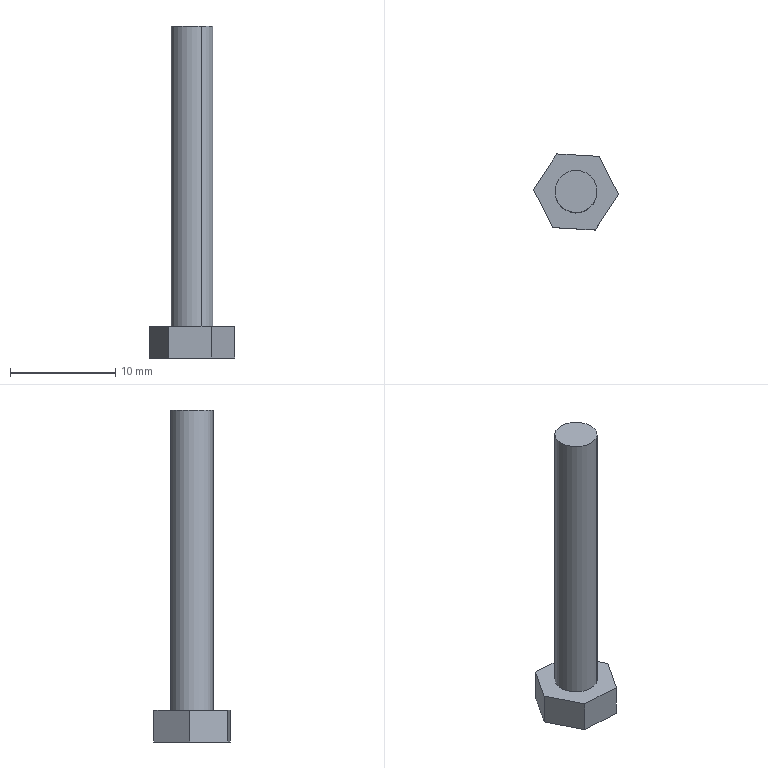Component | SolidWorks | 4Bolt-3 | 1 solid | 11 faces | box 8.07 x 7.22 x 31.5 mm | volume 485 mm3 | plane 9 | cylinder 2 | commonest cylinder face diameters 4 x2
STEP:
#1=COLOUR_RGB('',0.7922,0.8196,0.9333);
#2=FILL_AREA_STYLE_COLOUR('',#1);
#3=FILL_AREA_STYLE('',(#2));
#4=SURFACE_STYLE_FILL_AREA(#3);
#5=SURFACE_SIDE_STYLE('',(#4));
#6=SURFACE_STYLE_USAGE(.BOTH.,#5);
#7=PRESENTATION_STYLE_ASSIGNMENT((#6));
#8=CARTESIAN_POINT('',(4.312,4.161,2.255));
#9=VERTEX_POINT('',#8);
#10=CARTESIAN_POINT('',(4.241,4.302,2.255));
#11=VERTEX_POINT('',#10);
#12=CARTESIAN_POINT('',(4.277,4.231,2.255));
#13=DIRECTION('',(0.,0.,1.));
#14=DIRECTION('',(0.4489,-0.8936,0.));
#15=AXIS2_PLACEMENT_3D('',#12,#13,#14);
#16=CIRCLE('',#15,0.07874);
#17=EDGE_CURVE('',#9,#11,#16,.T.);
#18=ORIENTED_EDGE('',*,*,#17,.F.);
#19=CARTESIAN_POINT('',(4.312,4.161,1.133));
#20=VERTEX_POINT('',#19);
#21=CARTESIAN_POINT('',(4.312,4.161,2.255));
#22=DIRECTION('',(0.,0.,-1.));
#23=VECTOR('',#22,39.37);
#24=LINE('',#21,#23);
#25=EDGE_CURVE('',#9,#20,#24,.T.);
#26=ORIENTED_EDGE('',*,*,#25,.T.);
#27=CARTESIAN_POINT('',(4.241,4.302,1.133));
#28=VERTEX_POINT('',#27);
#29=CARTESIAN_POINT('',(4.277,4.231,1.133));
#30=DIRECTION('',(0.,0.,1.));
#31=DIRECTION('',(0.4489,-0.8936,0.));
#32=AXIS2_PLACEMENT_3D('',#29,#30,#31);
#33=CIRCLE('',#32,0.07874);
#34=EDGE_CURVE('',#20,#28,#33,.T.);
#35=ORIENTED_EDGE('',*,*,#34,.T.);
#36=CARTESIAN_POINT('',(4.241,4.302,2.255));
#37=DIRECTION('',(0.,0.,-1.));
#38=VECTOR('',#37,39.37);
#39=LINE('',#36,#38);
#40=EDGE_CURVE('',#11,#28,#39,.T.);
#41=ORIENTED_EDGE('',*,*,#40,.F.);
#42=EDGE_LOOP('',(#18,#26,#35,#41));
#43=FACE_OUTER_BOUND('',#42,.T.);
#44=CARTESIAN_POINT('',(4.277,4.231,2.255));
#45=DIRECTION('',(0.,0.,-1.));
#46=DIRECTION('',(-0.4489,0.8936,0.));
#47=AXIS2_PLACEMENT_3D('',#44,#45,#46);
#48=CYLINDRICAL_SURFACE('',#47,0.07874);
#49=ADVANCED_FACE('',(#43),#48,.T.);
#50=CARTESIAN_POINT('',(4.189,4.098,1.015));
#51=VERTEX_POINT('',#50);
#52=CARTESIAN_POINT('',(4.348,4.089,1.015));
#53=VERTEX_POINT('',#52);
#54=CARTESIAN_POINT('',(4.189,4.098,1.015));
#55=DIRECTION('',(0.9983,-0.05809,0.));
#56=VECTOR('',#55,39.37);
#57=LINE('',#54,#56);
#58=EDGE_CURVE('',#51,#53,#57,.T.);
#59=ORIENTED_EDGE('',*,*,#58,.T.);
#60=CARTESIAN_POINT('',(4.348,4.089,1.133));
#61=VERTEX_POINT('',#60);
#62=CARTESIAN_POINT('',(4.348,4.089,1.133));
#63=DIRECTION('',(0.,0.,-1.));
#64=VECTOR('',#63,39.37);
#65=LINE('',#62,#64);
#66=EDGE_CURVE('',#61,#53,#65,.T.);
#67=ORIENTED_EDGE('',*,*,#66,.F.);
#68=CARTESIAN_POINT('',(4.189,4.098,1.133));
#69=VERTEX_POINT('',#68);
#70=CARTESIAN_POINT('',(4.189,4.098,1.133));
#71=DIRECTION('',(0.9983,-0.05809,0.));
#72=VECTOR('',#71,39.37);
#73=LINE('',#70,#72);
#74=EDGE_CURVE('',#69,#61,#73,.T.);
#75=ORIENTED_EDGE('',*,*,#74,.F.);
#76=CARTESIAN_POINT('',(4.189,4.098,1.133));
#77=DIRECTION('',(0.,0.,-1.));
#78=VECTOR('',#77,39.37);
#79=LINE('',#76,#78);
#80=EDGE_CURVE('',#69,#51,#79,.T.);
#81=ORIENTED_EDGE('',*,*,#80,.T.);
#82=EDGE_LOOP('',(#59,#67,#75,#81));
#83=FACE_OUTER_BOUND('',#82,.T.);
#84=CARTESIAN_POINT('',(4.189,4.098,1.133));
#85=DIRECTION('',(0.05809,0.9983,0.));
#86=DIRECTION('',(-0.9983,0.05809,0.));
#87=AXIS2_PLACEMENT_3D('',#84,#85,#86);
#88=PLANE('',#87);
#89=ADVANCED_FACE('',(#83),#88,.F.);
#90=CARTESIAN_POINT('',(4.435,4.222,1.015));
#91=VERTEX_POINT('',#90);
#92=CARTESIAN_POINT('',(4.348,4.089,1.015));
#93=DIRECTION('',(0.5495,0.8355,0.));
#94=VECTOR('',#93,39.37);
#95=LINE('',#92,#94);
#96=EDGE_CURVE('',#53,#91,#95,.T.);
#97=ORIENTED_EDGE('',*,*,#96,.T.);
#98=CARTESIAN_POINT('',(4.435,4.222,1.133));
#99=VERTEX_POINT('',#98);
#100=CARTESIAN_POINT('',(4.435,4.222,1.133));
#101=DIRECTION('',(0.,0.,-1.));
#102=VECTOR('',#101,39.37);
#103=LINE('',#100,#102);
#104=EDGE_CURVE('',#99,#91,#103,.T.);
#105=ORIENTED_EDGE('',*,*,#104,.F.);
#106=CARTESIAN_POINT('',(4.348,4.089,1.133));
#107=DIRECTION('',(0.5495,0.8355,0.));
#108=VECTOR('',#107,39.37);
#109=LINE('',#106,#108);
#110=EDGE_CURVE('',#61,#99,#109,.T.);
#111=ORIENTED_EDGE('',*,*,#110,.F.);
#112=ORIENTED_EDGE('',*,*,#66,.T.);
#113=EDGE_LOOP('',(#97,#105,#111,#112));
#114=FACE_OUTER_BOUND('',#113,.T.);
#115=CARTESIAN_POINT('',(4.348,4.089,1.133));
#116=DIRECTION('',(-0.8355,0.5495,0.));
#117=DIRECTION('',(-0.5495,-0.8355,0.));
#118=AXIS2_PLACEMENT_3D('',#115,#116,#117);
#119=PLANE('',#118);
#120=ADVANCED_FACE('',(#114),#119,.F.);
#121=CARTESIAN_POINT('',(4.364,4.364,1.015));
#122=VERTEX_POINT('',#121);
#123=CARTESIAN_POINT('',(4.435,4.222,1.015));
#124=DIRECTION('',(-0.4489,0.8936,0.));
#125=VECTOR('',#124,39.37);
#126=LINE('',#123,#125);
#127=EDGE_CURVE('',#91,#122,#126,.T.);
#128=ORIENTED_EDGE('',*,*,#127,.T.);
#129=CARTESIAN_POINT('',(4.364,4.364,1.133));
#130=VERTEX_POINT('',#129);
#131=CARTESIAN_POINT('',(4.364,4.364,1.133));
#132=DIRECTION('',(0.,0.,-1.));
#133=VECTOR('',#132,39.37);
#134=LINE('',#131,#133);
#135=EDGE_CURVE('',#130,#122,#134,.T.);
#136=ORIENTED_EDGE('',*,*,#135,.F.);
#137=CARTESIAN_POINT('',(4.435,4.222,1.133));
#138=DIRECTION('',(-0.4489,0.8936,0.));
#139=VECTOR('',#138,39.37);
#140=LINE('',#137,#139);
#141=EDGE_CURVE('',#99,#130,#140,.T.);
#142=ORIENTED_EDGE('',*,*,#141,.F.);
#143=ORIENTED_EDGE('',*,*,#104,.T.);
#144=EDGE_LOOP('',(#128,#136,#142,#143));
#145=FACE_OUTER_BOUND('',#144,.T.);
#146=CARTESIAN_POINT('',(4.435,4.222,1.133));
#147=DIRECTION('',(-0.8936,-0.4489,0.));
#148=DIRECTION('',(0.,0.,-1.));
#149=AXIS2_PLACEMENT_3D('',#146,#147,#148);
#150=PLANE('',#149);
#151=ADVANCED_FACE('',(#145),#150,.F.);
#152=CARTESIAN_POINT('',(4.205,4.373,1.015));
#153=VERTEX_POINT('',#152);
#154=CARTESIAN_POINT('',(4.364,4.364,1.015));
#155=DIRECTION('',(-0.9983,0.05809,0.));
#156=VECTOR('',#155,39.37);
#157=LINE('',#154,#156);
#158=EDGE_CURVE('',#122,#153,#157,.T.);
#159=ORIENTED_EDGE('',*,*,#158,.T.);
#160=CARTESIAN_POINT('',(4.205,4.373,1.133));
#161=VERTEX_POINT('',#160);
#162=CARTESIAN_POINT('',(4.205,4.373,1.133));
#163=DIRECTION('',(0.,0.,-1.));
#164=VECTOR('',#163,39.37);
#165=LINE('',#162,#164);
#166=EDGE_CURVE('',#161,#153,#165,.T.);
#167=ORIENTED_EDGE('',*,*,#166,.F.);
#168=CARTESIAN_POINT('',(4.364,4.364,1.133));
#169=DIRECTION('',(-0.9983,0.05809,0.));
#170=VECTOR('',#169,39.37);
#171=LINE('',#168,#170);
#172=EDGE_CURVE('',#130,#161,#171,.T.);
#173=ORIENTED_EDGE('',*,*,#172,.F.);
#174=ORIENTED_EDGE('',*,*,#135,.T.);
#175=EDGE_LOOP('',(#159,#167,#173,#174));
#176=FACE_OUTER_BOUND('',#175,.T.);
#177=CARTESIAN_POINT('',(4.364,4.364,1.133));
#178=DIRECTION('',(-0.05809,-0.9983,0.));
#179=DIRECTION('',(0.9983,-0.05809,0.));
#180=AXIS2_PLACEMENT_3D('',#177,#178,#179);
#181=PLANE('',#180);
#182=ADVANCED_FACE('',(#176),#181,.F.);
#183=CARTESIAN_POINT('',(4.118,4.24,1.015));
#184=VERTEX_POINT('',#183);
#185=CARTESIAN_POINT('',(4.205,4.373,1.015));
#186=DIRECTION('',(-0.5495,-0.8355,0.));
#187=VECTOR('',#186,39.37);
#188=LINE('',#185,#187);
#189=EDGE_CURVE('',#153,#184,#188,.T.);
#190=ORIENTED_EDGE('',*,*,#189,.T.);
#191=CARTESIAN_POINT('',(4.118,4.24,1.133));
#192=VERTEX_POINT('',#191);
#193=CARTESIAN_POINT('',(4.118,4.24,1.133));
#194=DIRECTION('',(0.,0.,-1.));
#195=VECTOR('',#194,39.37);
#196=LINE('',#193,#195);
#197=EDGE_CURVE('',#192,#184,#196,.T.);
#198=ORIENTED_EDGE('',*,*,#197,.F.);
#199=CARTESIAN_POINT('',(4.205,4.373,1.133));
#200=DIRECTION('',(-0.5495,-0.8355,0.));
#201=VECTOR('',#200,39.37);
#202=LINE('',#199,#201);
#203=EDGE_CURVE('',#161,#192,#202,.T.);
#204=ORIENTED_EDGE('',*,*,#203,.F.);
#205=ORIENTED_EDGE('',*,*,#166,.T.);
#206=EDGE_LOOP('',(#190,#198,#204,#205));
#207=FACE_OUTER_BOUND('',#206,.T.);
#208=CARTESIAN_POINT('',(4.205,4.373,1.133));
#209=DIRECTION('',(0.8355,-0.5495,0.));
#210=DIRECTION('',(0.5495,0.8355,0.));
#211=AXIS2_PLACEMENT_3D('',#208,#209,#210);
#212=PLANE('',#211);
#213=ADVANCED_FACE('',(#207),#212,.F.);
#214=CARTESIAN_POINT('',(4.118,4.24,1.015));
#215=DIRECTION('',(0.4489,-0.8936,0.));
#216=VECTOR('',#215,39.37);
#217=LINE('',#214,#216);
#218=EDGE_CURVE('',#184,#51,#217,.T.);
#219=ORIENTED_EDGE('',*,*,#218,.T.);
#220=ORIENTED_EDGE('',*,*,#80,.F.);
#221=CARTESIAN_POINT('',(4.118,4.24,1.133));
#222=DIRECTION('',(0.4489,-0.8936,0.));
#223=VECTOR('',#222,39.37);
#224=LINE('',#221,#223);
#225=EDGE_CURVE('',#192,#69,#224,.T.);
#226=ORIENTED_EDGE('',*,*,#225,.F.);
#227=ORIENTED_EDGE('',*,*,#197,.T.);
#228=EDGE_LOOP('',(#219,#220,#226,#227));
#229=FACE_OUTER_BOUND('',#228,.T.);
#230=CARTESIAN_POINT('',(4.118,4.24,1.133));
#231=DIRECTION('',(0.8936,0.4489,0.));
#232=DIRECTION('',(-0.4489,0.8936,0.));
#233=AXIS2_PLACEMENT_3D('',#230,#231,#232);
#234=PLANE('',#233);
#235=ADVANCED_FACE('',(#229),#234,.F.);
#236=CARTESIAN_POINT('',(4.277,4.231,1.133));
#237=DIRECTION('',(0.,0.,1.));
#238=DIRECTION('',(0.4489,-0.8936,0.));
#239=AXIS2_PLACEMENT_3D('',#236,#237,#238);
#240=CIRCLE('',#239,0.07874);
#241=EDGE_CURVE('',#28,#20,#240,.T.);
#242=ORIENTED_EDGE('',*,*,#241,.F.);
#243=ORIENTED_EDGE('',*,*,#34,.F.);
#244=EDGE_LOOP('',(#242,#243));
#245=FACE_BOUND('',#244,.T.);
#246=ORIENTED_EDGE('',*,*,#74,.T.);
#247=ORIENTED_EDGE('',*,*,#110,.T.);
#248=ORIENTED_EDGE('',*,*,#141,.T.);
#249=ORIENTED_EDGE('',*,*,#172,.T.);
#250=ORIENTED_EDGE('',*,*,#203,.T.);
#251=ORIENTED_EDGE('',*,*,#225,.T.);
#252=EDGE_LOOP('',(#246,#247,#248,#249,#250,#251));
#253=FACE_OUTER_BOUND('',#252,.T.);
#254=CARTESIAN_POINT('',(4.277,4.231,1.133));
#255=DIRECTION('',(0.,0.,1.));
#256=DIRECTION('',(0.4489,-0.8936,0.));
#257=AXIS2_PLACEMENT_3D('',#254,#255,#256);
#258=PLANE('',#257);
#259=ADVANCED_FACE('',(#245,#253),#258,.T.);
#260=ORIENTED_EDGE('',*,*,#58,.F.);
#261=ORIENTED_EDGE('',*,*,#218,.F.);
#262=ORIENTED_EDGE('',*,*,#189,.F.);
#263=ORIENTED_EDGE('',*,*,#158,.F.);
#264=ORIENTED_EDGE('',*,*,#127,.F.);
#265=ORIENTED_EDGE('',*,*,#96,.F.);
#266=EDGE_LOOP('',(#260,#261,#262,#263,#264,#265));
#267=FACE_OUTER_BOUND('',#266,.T.);
#268=CARTESIAN_POINT('',(4.277,4.231,1.015));
#269=DIRECTION('',(0.,0.,1.));
#270=DIRECTION('',(0.4489,-0.8936,0.));
#271=AXIS2_PLACEMENT_3D('',#268,#269,#270);
#272=PLANE('',#271);
#273=ADVANCED_FACE('',(#267),#272,.F.);
#274=ORIENTED_EDGE('',*,*,#25,.F.);
#275=CARTESIAN_POINT('',(4.277,4.231,2.255));
#276=DIRECTION('',(0.,0.,1.));
#277=DIRECTION('',(0.4489,-0.8936,0.));
#278=AXIS2_PLACEMENT_3D('',#275,#276,#277);
#279=CIRCLE('',#278,0.07874);
#280=EDGE_CURVE('',#11,#9,#279,.T.);
#281=ORIENTED_EDGE('',*,*,#280,.F.);
#282=ORIENTED_EDGE('',*,*,#40,.T.);
#283=ORIENTED_EDGE('',*,*,#241,.T.);
#284=EDGE_LOOP('',(#274,#281,#282,#283));
#285=FACE_OUTER_BOUND('',#284,.T.);
#286=CARTESIAN_POINT('',(4.277,4.231,2.255));
#287=DIRECTION('',(0.,0.,-1.));
#288=DIRECTION('',(-0.4489,0.8936,0.));
#289=AXIS2_PLACEMENT_3D('',#286,#287,#288);
#290=CYLINDRICAL_SURFACE('',#289,0.07874);
#291=ADVANCED_FACE('',(#285),#290,.T.);
#292=ORIENTED_EDGE('',*,*,#280,.T.);
#293=ORIENTED_EDGE('',*,*,#17,.T.);
#294=EDGE_LOOP('',(#292,#293));
#295=FACE_OUTER_BOUND('',#294,.T.);
#296=CARTESIAN_POINT('',(4.277,4.231,2.255));
#297=DIRECTION('',(0.,0.,1.));
#298=DIRECTION('',(0.4489,-0.8936,0.));
#299=AXIS2_PLACEMENT_3D('',#296,#297,#298);
#300=PLANE('',#299);
#301=ADVANCED_FACE('',(#295),#300,.T.);
#302=CLOSED_SHELL('',(#49,#89,#120,#151,#182,#213,#235,#259,#273,#291,#301));
#303=MANIFOLD_SOLID_BREP('',#302);
#304=STYLED_ITEM('',(#7),#303);
#305=(LENGTH_UNIT()NAMED_UNIT(*)SI_UNIT($,.METRE.));
#306=LENGTH_MEASURE_WITH_UNIT(LENGTH_MEASURE(0.0254),#305);
#307=DIMENSIONAL_EXPONENTS(1.,0.,0.,0.,0.,0.,0.);
#308=(CONVERSION_BASED_UNIT('',#306)LENGTH_UNIT()NAMED_UNIT(#307));
#309=UNCERTAINTY_MEASURE_WITH_UNIT(LENGTH_MEASURE(0.00001),#308,'','');
#310=(NAMED_UNIT(*)PLANE_ANGLE_UNIT()SI_UNIT($,.RADIAN.));
#311=(NAMED_UNIT(*)SI_UNIT($,.STERADIAN.)SOLID_ANGLE_UNIT());
#312=(GEOMETRIC_REPRESENTATION_CONTEXT(3)GLOBAL_UNCERTAINTY_ASSIGNED_CONTEXT((#309))GLOBAL_UNIT_ASSIGNED_CONTEXT((#308,#310,#311))REPRESENTATION_CONTEXT('',''));
#313=MECHANICAL_DESIGN_GEOMETRIC_PRESENTATION_REPRESENTATION('',(#304),#312);
#314=CARTESIAN_POINT('',(0.,0.,0.));
#315=DIRECTION('',(0.,0.,1.));
#316=DIRECTION('',(1.,0.,0.));
#317=AXIS2_PLACEMENT_3D('',#314,#315,#316);
#318=(LENGTH_UNIT()NAMED_UNIT(*)SI_UNIT($,.METRE.));
#319=LENGTH_MEASURE_WITH_UNIT(LENGTH_MEASURE(0.0254),#318);
#320=DIMENSIONAL_EXPONENTS(1.,0.,0.,0.,0.,0.,0.);
#321=(CONVERSION_BASED_UNIT('',#319)LENGTH_UNIT()NAMED_UNIT(#320));
#322=UNCERTAINTY_MEASURE_WITH_UNIT(LENGTH_MEASURE(0.00001),#321,'','');
#323=(NAMED_UNIT(*)PLANE_ANGLE_UNIT()SI_UNIT($,.RADIAN.));
#324=(NAMED_UNIT(*)SI_UNIT($,.STERADIAN.)SOLID_ANGLE_UNIT());
#325=(GEOMETRIC_REPRESENTATION_CONTEXT(3)GLOBAL_UNCERTAINTY_ASSIGNED_CONTEXT((#322))GLOBAL_UNIT_ASSIGNED_CONTEXT((#321,#323,#324))REPRESENTATION_CONTEXT('',''));
#326=ADVANCED_BREP_SHAPE_REPRESENTATION('',(#303,#317),#325);
#327=PRESENTATION_LAYER_ASSIGNMENT('','',(#304));